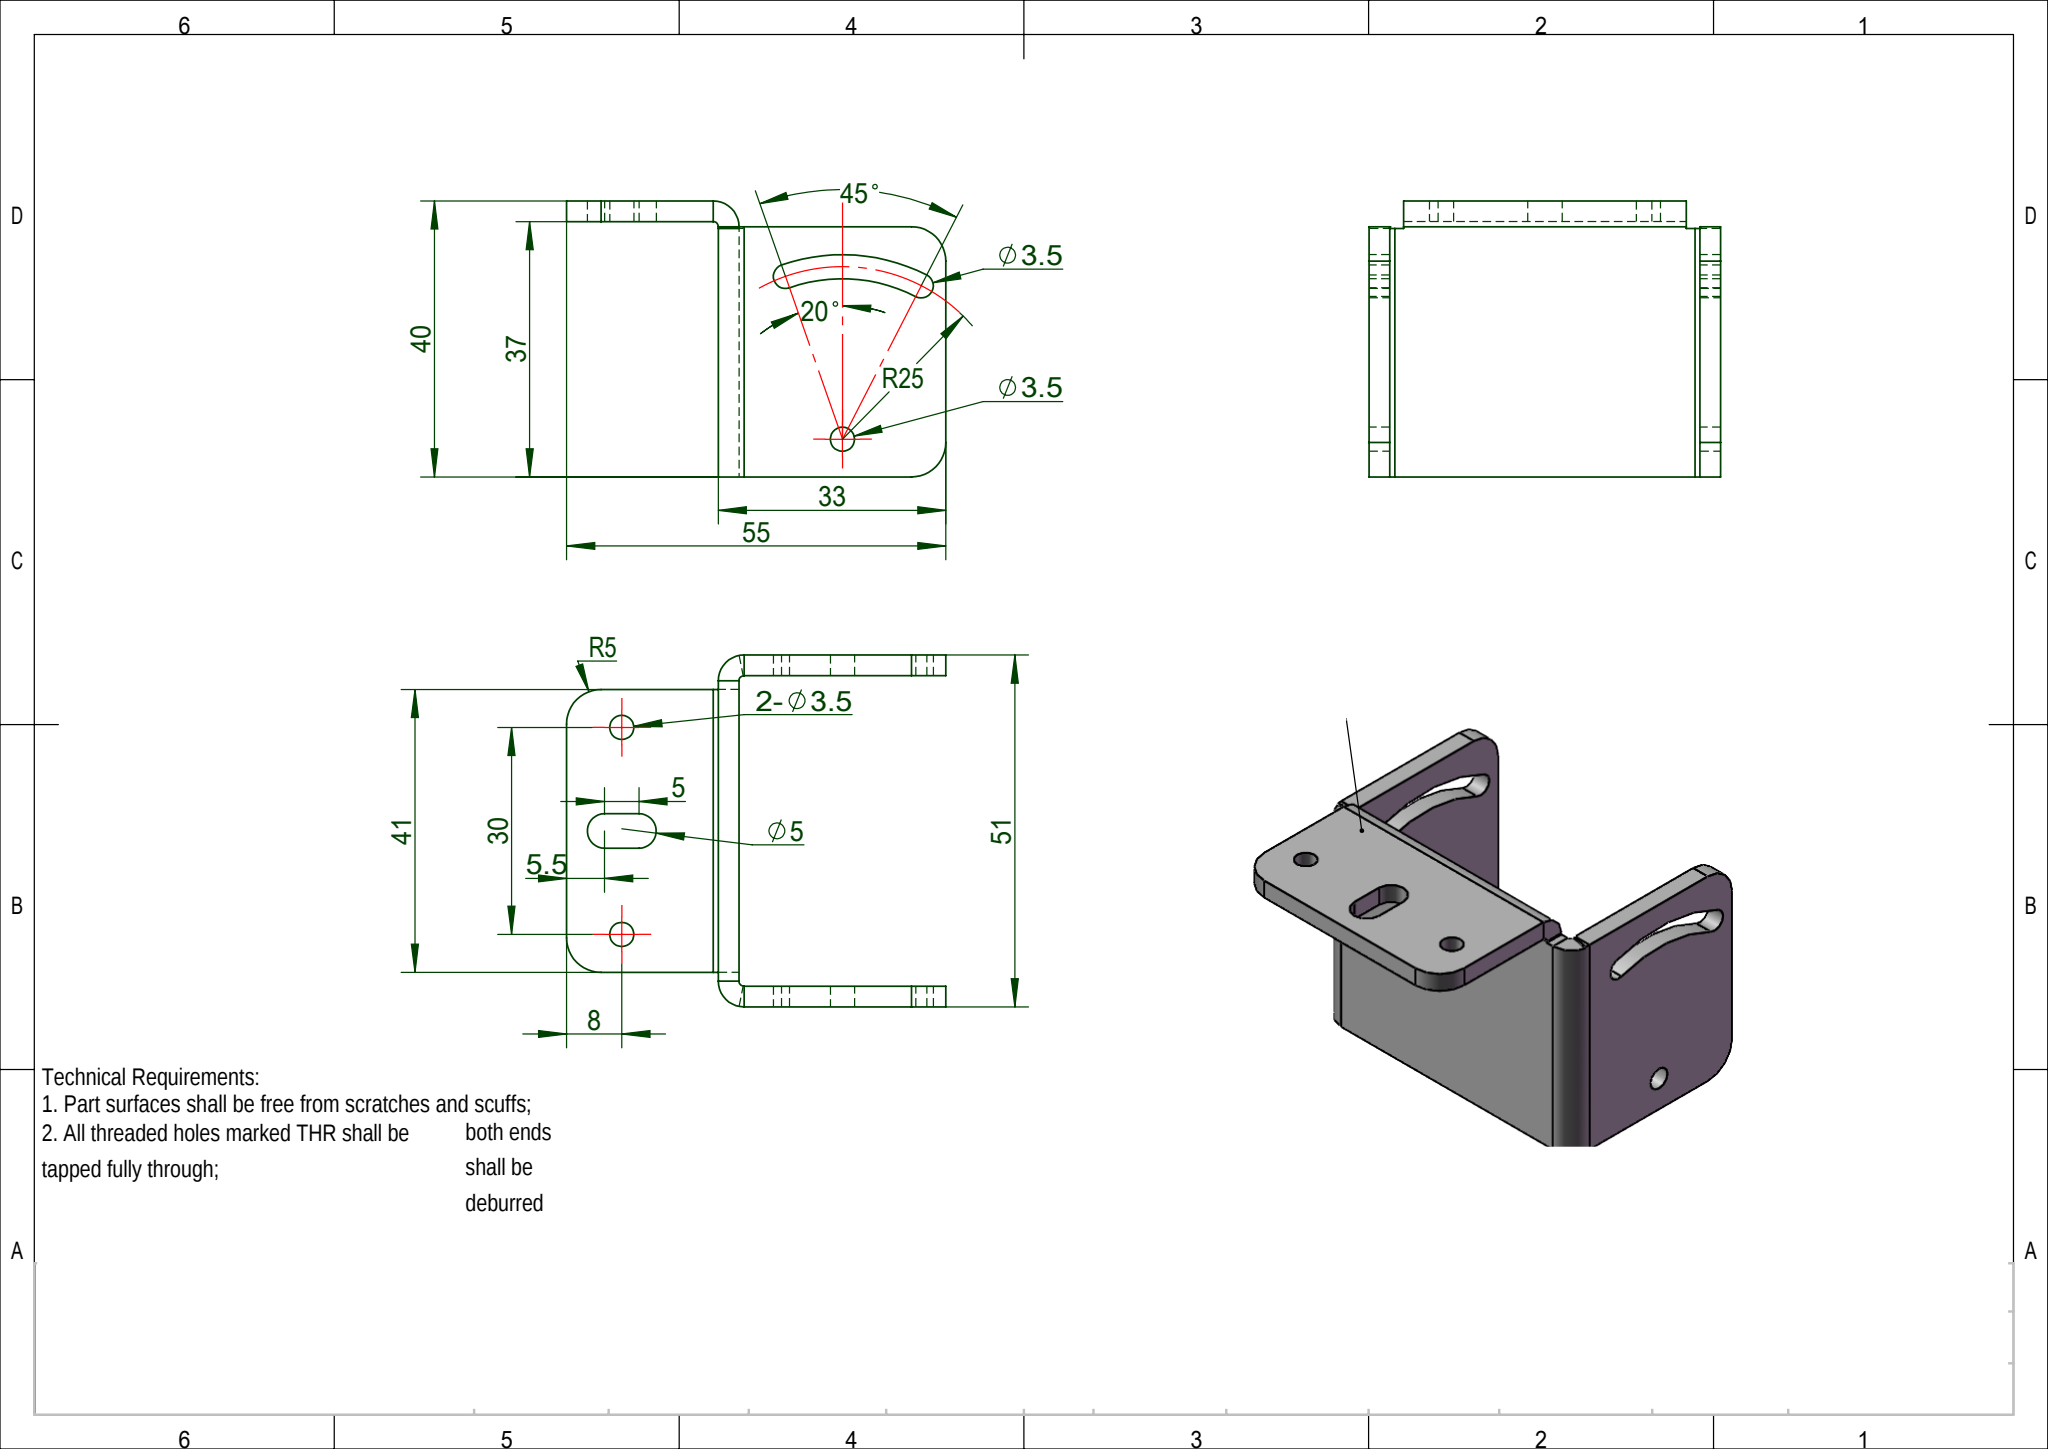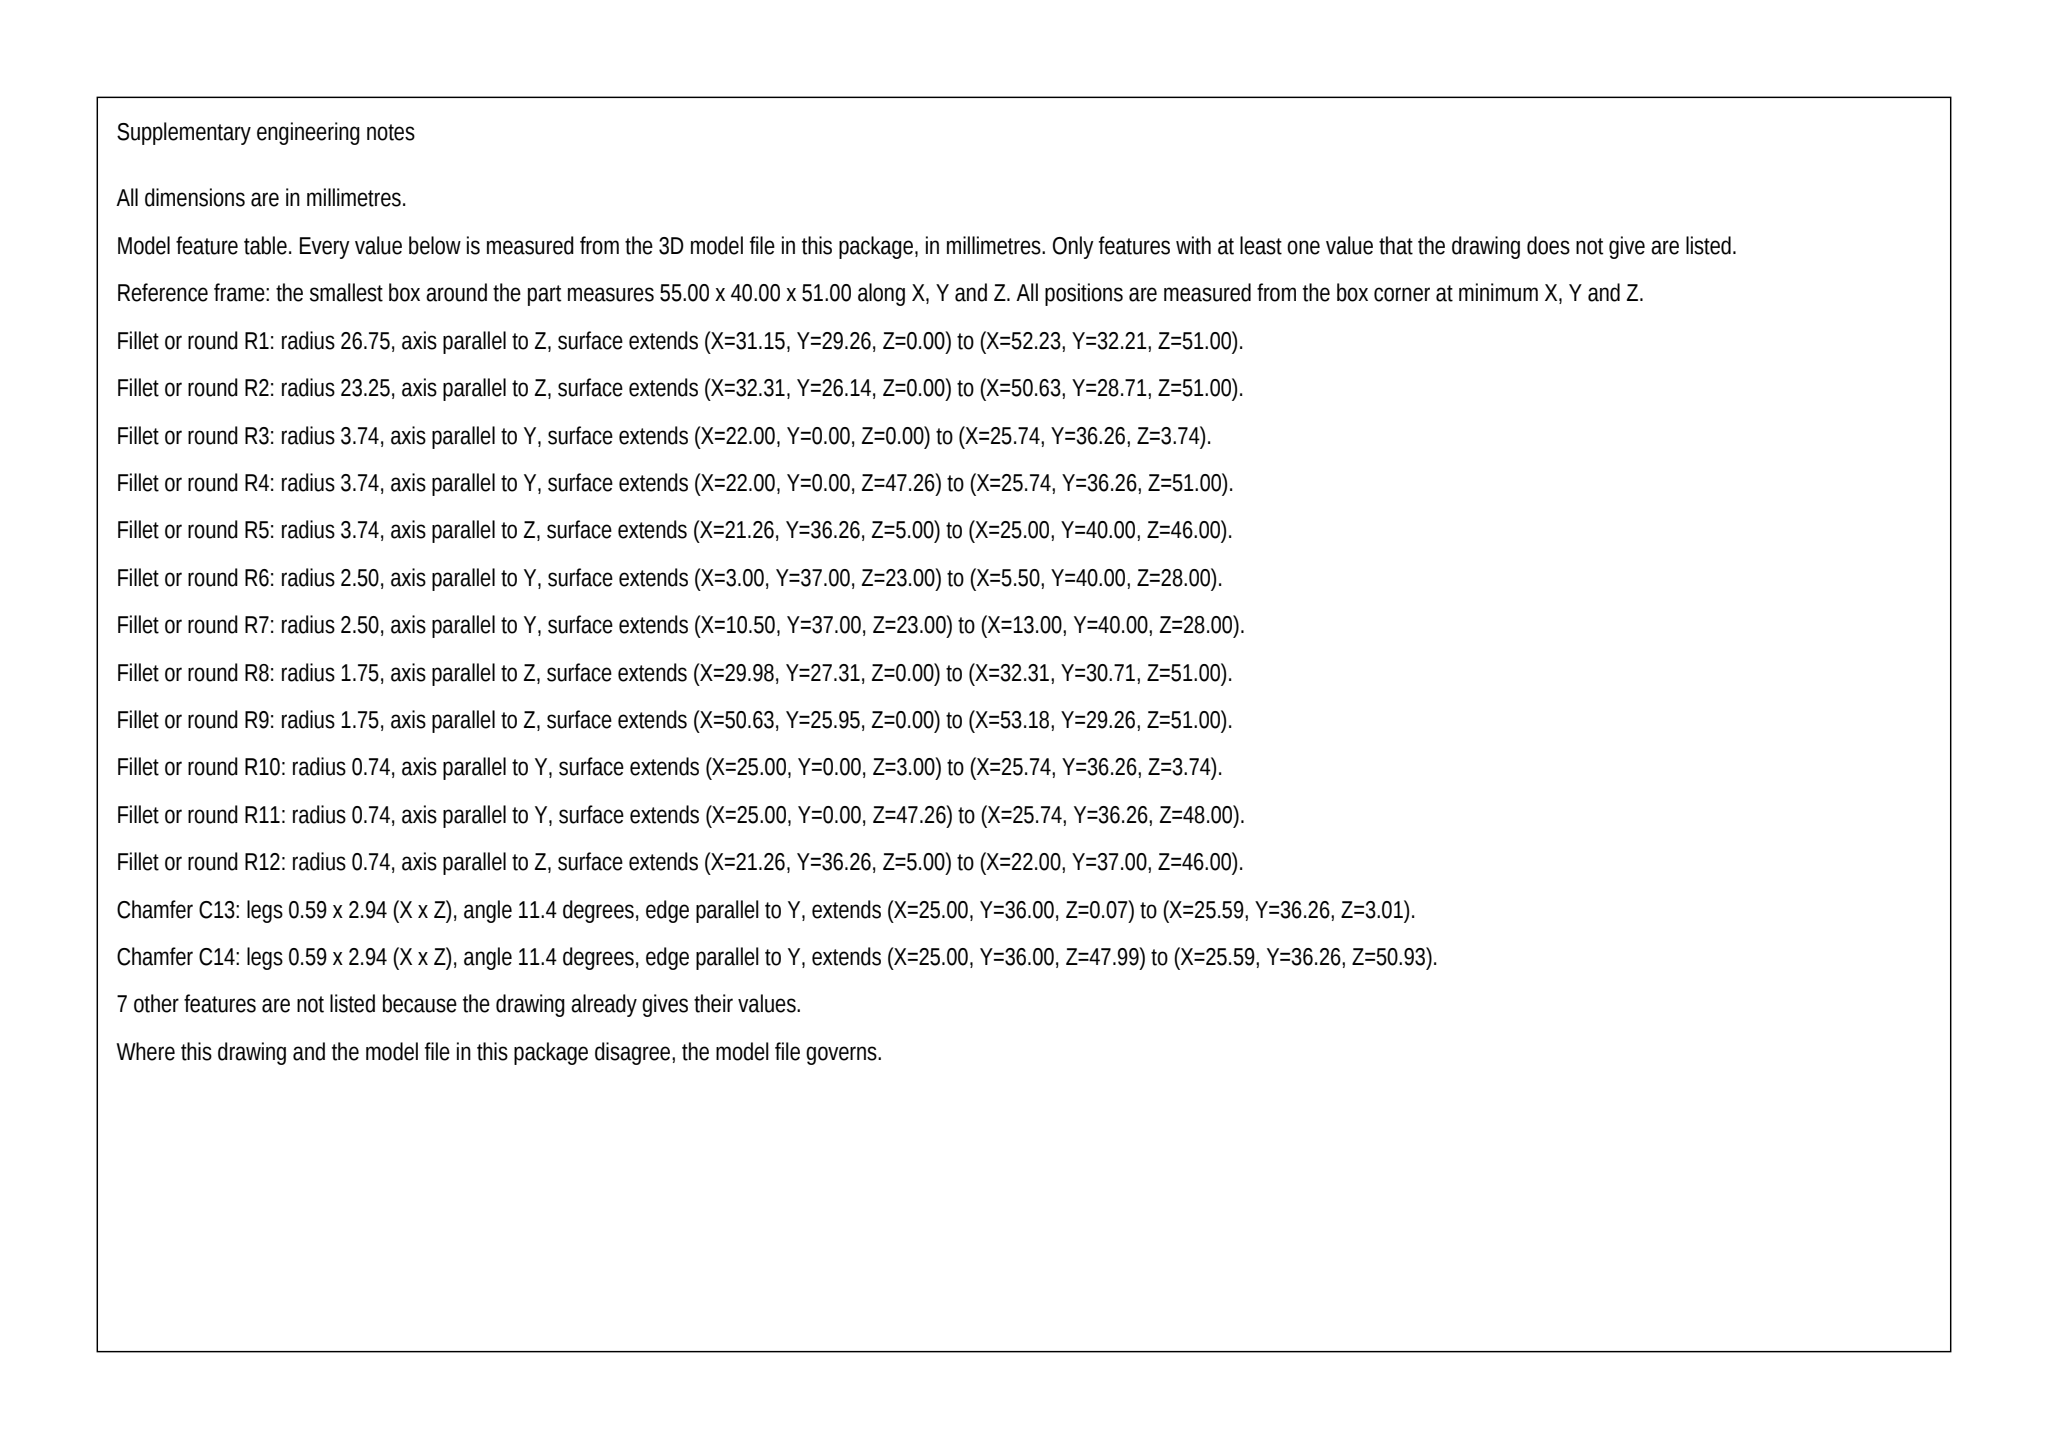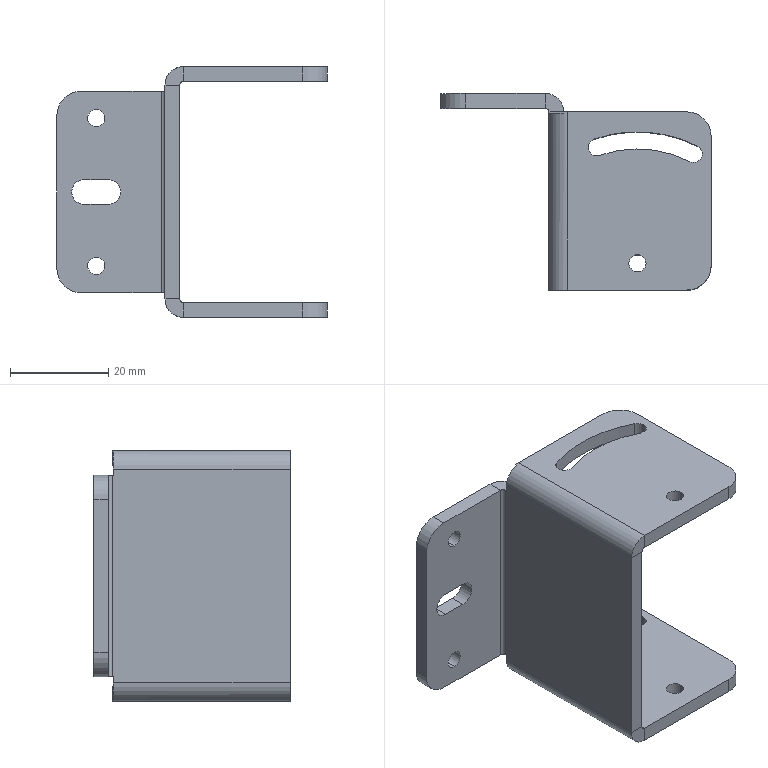Part | SolidWorks | mm | 1 solid | 66 faces | box 55 x 40 x 51 mm | volume 14078 mm3 | plane 34 | cylinder 32 | commonest cylinder face diameters 3.5 x14 10 x6 7.473 x3 1.473 x3 5 x2 53.5 x2 46.5 x2